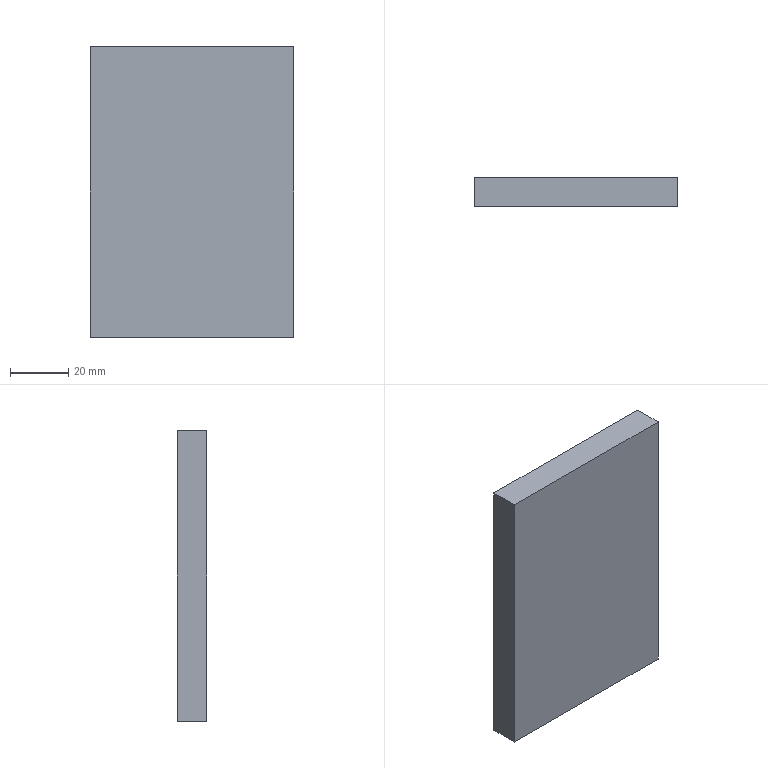Component | SolidWorks | THK-A1014BothSidesReinforcementPlate-2 | 1 solid | 6 faces | box 70 x 10 x 100 mm | volume 70000 mm3 | plane 6 | material Q235A
build123d program:
from build123d import *

# Parameters (mm, degrees)
SKETCH1_W           = 70
SKETCH1_H           = 10
BOSS_EXTRUDE1_DEPTH = 50


with BuildPart() as part:
    # Sketch1 → Boss-Extrude1 (new, symmetric)
    with BuildSketch(Plane(origin=(0, 0, 0), x_dir=(-1, 0, 0), z_dir=(0, 0, -1))):
        Rectangle(SKETCH1_W, SKETCH1_H)
    extrude(amount=BOSS_EXTRUDE1_DEPTH, both=True)


solid = part.part

# Placed as in the assembly
solid = solid.moved(Location((-165, -50, -321), (0, 0, 0)))
STEP:
#1=COLOUR_RGB('',0.7922,0.8196,0.9333);
#2=FILL_AREA_STYLE_COLOUR('',#1);
#3=FILL_AREA_STYLE('',(#2));
#4=SURFACE_STYLE_FILL_AREA(#3);
#5=SURFACE_SIDE_STYLE('',(#4));
#6=SURFACE_STYLE_USAGE(.BOTH.,#5);
#7=PRESENTATION_STYLE_ASSIGNMENT((#6));
#8=CARTESIAN_POINT('',(-7.874,-1.772,-14.606));
#9=VERTEX_POINT('',#8);
#10=CARTESIAN_POINT('',(-7.874,-2.165,-14.606));
#11=VERTEX_POINT('',#10);
#12=CARTESIAN_POINT('',(-7.874,-2.165,-14.606));
#13=DIRECTION('',(0.,-1.,0.));
#14=VECTOR('',#13,39.37);
#15=LINE('',#12,#14);
#16=EDGE_CURVE('',#9,#11,#15,.T.);
#17=ORIENTED_EDGE('',*,*,#16,.T.);
#18=CARTESIAN_POINT('',(-7.874,-2.165,-10.669));
#19=VERTEX_POINT('',#18);
#20=CARTESIAN_POINT('',(-7.874,-2.165,-10.669));
#21=DIRECTION('',(0.,0.,-1.));
#22=VECTOR('',#21,39.37);
#23=LINE('',#20,#22);
#24=EDGE_CURVE('',#19,#11,#23,.T.);
#25=ORIENTED_EDGE('',*,*,#24,.F.);
#26=CARTESIAN_POINT('',(-7.874,-1.772,-10.669));
#27=VERTEX_POINT('',#26);
#28=CARTESIAN_POINT('',(-7.874,-2.165,-10.669));
#29=DIRECTION('',(0.,-1.,0.));
#30=VECTOR('',#29,39.37);
#31=LINE('',#28,#30);
#32=EDGE_CURVE('',#27,#19,#31,.T.);
#33=ORIENTED_EDGE('',*,*,#32,.F.);
#34=CARTESIAN_POINT('',(-7.874,-1.772,-10.669));
#35=DIRECTION('',(0.,0.,-1.));
#36=VECTOR('',#35,39.37);
#37=LINE('',#34,#36);
#38=EDGE_CURVE('',#27,#9,#37,.T.);
#39=ORIENTED_EDGE('',*,*,#38,.T.);
#40=EDGE_LOOP('',(#17,#25,#33,#39));
#41=FACE_OUTER_BOUND('',#40,.T.);
#42=CARTESIAN_POINT('',(-7.874,-2.165,-10.669));
#43=DIRECTION('',(1.,0.,0.));
#44=DIRECTION('',(0.,0.,-1.));
#45=AXIS2_PLACEMENT_3D('',#42,#43,#44);
#46=PLANE('',#45);
#47=ADVANCED_FACE('',(#41),#46,.F.);
#48=CARTESIAN_POINT('',(-5.118,-2.165,-14.606));
#49=VERTEX_POINT('',#48);
#50=CARTESIAN_POINT('',(-5.118,-2.165,-14.606));
#51=DIRECTION('',(1.,0.,-0.));
#52=VECTOR('',#51,39.37);
#53=LINE('',#50,#52);
#54=EDGE_CURVE('',#11,#49,#53,.T.);
#55=ORIENTED_EDGE('',*,*,#54,.T.);
#56=CARTESIAN_POINT('',(-5.118,-2.165,-10.669));
#57=VERTEX_POINT('',#56);
#58=CARTESIAN_POINT('',(-5.118,-2.165,-10.669));
#59=DIRECTION('',(0.,0.,-1.));
#60=VECTOR('',#59,39.37);
#61=LINE('',#58,#60);
#62=EDGE_CURVE('',#57,#49,#61,.T.);
#63=ORIENTED_EDGE('',*,*,#62,.F.);
#64=CARTESIAN_POINT('',(-5.118,-2.165,-10.669));
#65=DIRECTION('',(1.,0.,-0.));
#66=VECTOR('',#65,39.37);
#67=LINE('',#64,#66);
#68=EDGE_CURVE('',#19,#57,#67,.T.);
#69=ORIENTED_EDGE('',*,*,#68,.F.);
#70=ORIENTED_EDGE('',*,*,#24,.T.);
#71=EDGE_LOOP('',(#55,#63,#69,#70));
#72=FACE_OUTER_BOUND('',#71,.T.);
#73=CARTESIAN_POINT('',(-5.118,-2.165,-10.669));
#74=DIRECTION('',(-0.,1.,-0.));
#75=DIRECTION('',(1.,0.,-0.));
#76=AXIS2_PLACEMENT_3D('',#73,#74,#75);
#77=PLANE('',#76);
#78=ADVANCED_FACE('',(#72),#77,.F.);
#79=CARTESIAN_POINT('',(-5.118,-1.772,-14.606));
#80=VERTEX_POINT('',#79);
#81=CARTESIAN_POINT('',(-5.118,-2.165,-14.606));
#82=DIRECTION('',(0.,1.,-0.));
#83=VECTOR('',#82,39.37);
#84=LINE('',#81,#83);
#85=EDGE_CURVE('',#49,#80,#84,.T.);
#86=ORIENTED_EDGE('',*,*,#85,.T.);
#87=CARTESIAN_POINT('',(-5.118,-1.772,-10.669));
#88=VERTEX_POINT('',#87);
#89=CARTESIAN_POINT('',(-5.118,-1.772,-10.669));
#90=DIRECTION('',(0.,0.,-1.));
#91=VECTOR('',#90,39.37);
#92=LINE('',#89,#91);
#93=EDGE_CURVE('',#88,#80,#92,.T.);
#94=ORIENTED_EDGE('',*,*,#93,.F.);
#95=CARTESIAN_POINT('',(-5.118,-2.165,-10.669));
#96=DIRECTION('',(0.,1.,-0.));
#97=VECTOR('',#96,39.37);
#98=LINE('',#95,#97);
#99=EDGE_CURVE('',#57,#88,#98,.T.);
#100=ORIENTED_EDGE('',*,*,#99,.F.);
#101=ORIENTED_EDGE('',*,*,#62,.T.);
#102=EDGE_LOOP('',(#86,#94,#100,#101));
#103=FACE_OUTER_BOUND('',#102,.T.);
#104=CARTESIAN_POINT('',(-5.118,-2.165,-10.669));
#105=DIRECTION('',(-1.,0.,0.));
#106=DIRECTION('',(0.,0.,1.));
#107=AXIS2_PLACEMENT_3D('',#104,#105,#106);
#108=PLANE('',#107);
#109=ADVANCED_FACE('',(#103),#108,.F.);
#110=CARTESIAN_POINT('',(-5.118,-1.772,-14.606));
#111=DIRECTION('',(-1.,-0.,0.));
#112=VECTOR('',#111,39.37);
#113=LINE('',#110,#112);
#114=EDGE_CURVE('',#80,#9,#113,.T.);
#115=ORIENTED_EDGE('',*,*,#114,.T.);
#116=ORIENTED_EDGE('',*,*,#38,.F.);
#117=CARTESIAN_POINT('',(-5.118,-1.772,-10.669));
#118=DIRECTION('',(-1.,-0.,0.));
#119=VECTOR('',#118,39.37);
#120=LINE('',#117,#119);
#121=EDGE_CURVE('',#88,#27,#120,.T.);
#122=ORIENTED_EDGE('',*,*,#121,.F.);
#123=ORIENTED_EDGE('',*,*,#93,.T.);
#124=EDGE_LOOP('',(#115,#116,#122,#123));
#125=FACE_OUTER_BOUND('',#124,.T.);
#126=CARTESIAN_POINT('',(-5.118,-1.772,-10.669));
#127=DIRECTION('',(0.,-1.,0.));
#128=DIRECTION('',(-1.,-0.,0.));
#129=AXIS2_PLACEMENT_3D('',#126,#127,#128);
#130=PLANE('',#129);
#131=ADVANCED_FACE('',(#125),#130,.F.);
#132=ORIENTED_EDGE('',*,*,#32,.T.);
#133=ORIENTED_EDGE('',*,*,#68,.T.);
#134=ORIENTED_EDGE('',*,*,#99,.T.);
#135=ORIENTED_EDGE('',*,*,#121,.T.);
#136=EDGE_LOOP('',(#132,#133,#134,#135));
#137=FACE_OUTER_BOUND('',#136,.T.);
#138=CARTESIAN_POINT('',(-6.496,-1.969,-10.669));
#139=DIRECTION('',(0.,0.,1.));
#140=DIRECTION('',(1.,0.,0.));
#141=AXIS2_PLACEMENT_3D('',#138,#139,#140);
#142=PLANE('',#141);
#143=ADVANCED_FACE('',(#137),#142,.T.);
#144=ORIENTED_EDGE('',*,*,#16,.F.);
#145=ORIENTED_EDGE('',*,*,#114,.F.);
#146=ORIENTED_EDGE('',*,*,#85,.F.);
#147=ORIENTED_EDGE('',*,*,#54,.F.);
#148=EDGE_LOOP('',(#144,#145,#146,#147));
#149=FACE_OUTER_BOUND('',#148,.T.);
#150=CARTESIAN_POINT('',(-6.496,-1.969,-14.606));
#151=DIRECTION('',(0.,0.,1.));
#152=DIRECTION('',(1.,0.,0.));
#153=AXIS2_PLACEMENT_3D('',#150,#151,#152);
#154=PLANE('',#153);
#155=ADVANCED_FACE('',(#149),#154,.F.);
#156=CLOSED_SHELL('',(#47,#78,#109,#131,#143,#155));
#157=MANIFOLD_SOLID_BREP('',#156);
#158=STYLED_ITEM('',(#7),#157);
#159=(LENGTH_UNIT()NAMED_UNIT(*)SI_UNIT($,.METRE.));
#160=LENGTH_MEASURE_WITH_UNIT(LENGTH_MEASURE(0.0254),#159);
#161=DIMENSIONAL_EXPONENTS(1.,0.,0.,0.,0.,0.,0.);
#162=(CONVERSION_BASED_UNIT('',#160)LENGTH_UNIT()NAMED_UNIT(#161));
#163=UNCERTAINTY_MEASURE_WITH_UNIT(LENGTH_MEASURE(0.00001),#162,'','');
#164=(NAMED_UNIT(*)PLANE_ANGLE_UNIT()SI_UNIT($,.RADIAN.));
#165=(NAMED_UNIT(*)SI_UNIT($,.STERADIAN.)SOLID_ANGLE_UNIT());
#166=(GEOMETRIC_REPRESENTATION_CONTEXT(3)GLOBAL_UNCERTAINTY_ASSIGNED_CONTEXT((#163))GLOBAL_UNIT_ASSIGNED_CONTEXT((#162,#164,#165))REPRESENTATION_CONTEXT('',''));
#167=MECHANICAL_DESIGN_GEOMETRIC_PRESENTATION_REPRESENTATION('',(#158),#166);
#168=PRESENTATION_LAYER_ASSIGNMENT('','',(#158));
#169=CARTESIAN_POINT('',(0.,0.,0.));
#170=DIRECTION('',(0.,0.,1.));
#171=DIRECTION('',(1.,0.,0.));
#172=AXIS2_PLACEMENT_3D('',#169,#170,#171);
#173=(LENGTH_UNIT()NAMED_UNIT(*)SI_UNIT($,.METRE.));
#174=LENGTH_MEASURE_WITH_UNIT(LENGTH_MEASURE(0.0254),#173);
#175=DIMENSIONAL_EXPONENTS(1.,0.,0.,0.,0.,0.,0.);
#176=(CONVERSION_BASED_UNIT('',#174)LENGTH_UNIT()NAMED_UNIT(#175));
#177=UNCERTAINTY_MEASURE_WITH_UNIT(LENGTH_MEASURE(0.00001),#176,'','');
#178=(NAMED_UNIT(*)PLANE_ANGLE_UNIT()SI_UNIT($,.RADIAN.));
#179=(NAMED_UNIT(*)SI_UNIT($,.STERADIAN.)SOLID_ANGLE_UNIT());
#180=(GEOMETRIC_REPRESENTATION_CONTEXT(3)GLOBAL_UNCERTAINTY_ASSIGNED_CONTEXT((#177))GLOBAL_UNIT_ASSIGNED_CONTEXT((#176,#178,#179))REPRESENTATION_CONTEXT('',''));
#181=ADVANCED_BREP_SHAPE_REPRESENTATION('',(#157,#172),#180);